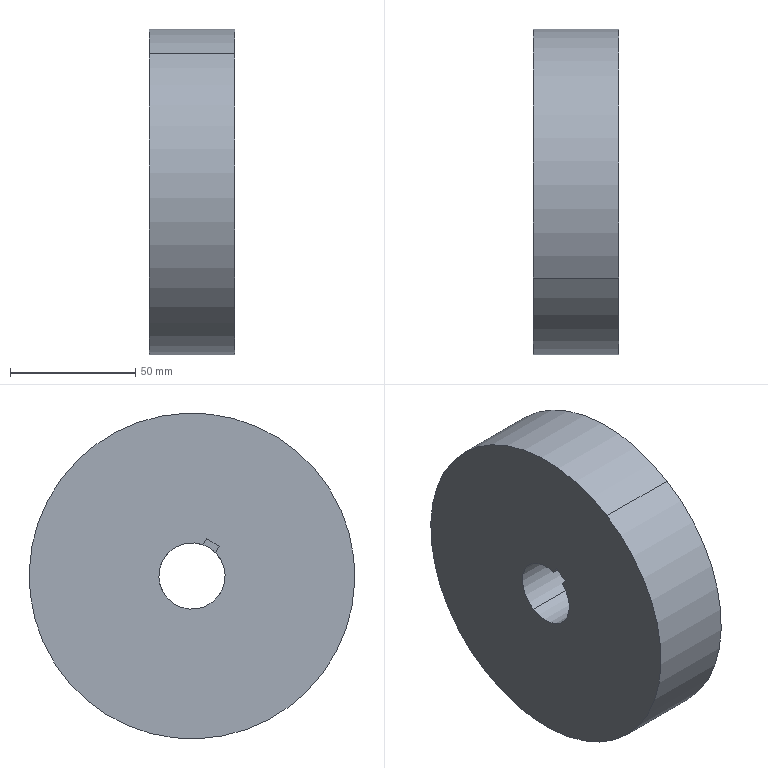Component | SolidWorks | Handwheel-1 | 1 solid | 13 faces | box 34 x 130 x 130 mm | volume 431777 mm3 | plane 7 | cylinder 6 | commonest cylinder face diameters 10 x2 26.469 x2 130 x2
build123d program:
from build123d import *

# Parameters (mm, degrees)
SKETCH1_R           = 65
SKETCH1_R_2         = 13.235
BOSS_EXTRUDE1_DEPTH = 34
SKETCH2_R           = 5
CUT_EXTRUDE1_DEPTH  = 8
CUT_EXTRUDE2_START  = -23
CUT_EXTRUDE2_DEPTH  = 11


with BuildPart() as part:
    # Sketch1 → Boss-Extrude1 (new body)
    with BuildSketch(Plane.XY):
        with Locations((15, 150)):
            Circle(SKETCH1_R)
        with Locations((15, 150)):
            Circle(SKETCH1_R_2, mode=Mode.SUBTRACT)
    extrude(amount=BOSS_EXTRUDE1_DEPTH)

    # Sketch2 → Cut-Extrude1 (cut)
    with BuildSketch(Plane.XY.offset(34)):
        with Locations((15, 199.291)):
            Circle(SKETCH2_R)
    extrude(amount=-CUT_EXTRUDE1_DEPTH, mode=Mode.SUBTRACT)

    # Sketch3 → Cut-Extrude2 (cut)
    with BuildSketch(Plane.XY.offset(34).offset(CUT_EXTRUDE2_START)):
        Polygon((2.855, 152.957), (-0.8059, 152.957), (-0.8059, 147.031), (2.855, 147.043), align=None)
    extrude(amount=-CUT_EXTRUDE2_DEPTH, mode=Mode.SUBTRACT)


solid = part.part

# Placed as in the assembly
solid = solid.moved(Location((133.63, 14.821, -81.721), (31.981, 90, 0)))
STEP:
#1=COLOUR_RGB('',0.7922,0.8196,0.9333);
#2=FILL_AREA_STYLE_COLOUR('',#1);
#3=FILL_AREA_STYLE('',(#2));
#4=SURFACE_STYLE_FILL_AREA(#3);
#5=SURFACE_SIDE_STYLE('',(#4));
#6=SURFACE_STYLE_USAGE(.BOTH.,#5);
#7=PRESENTATION_STYLE_ASSIGNMENT((#6));
#8=CARTESIAN_POINT('',(6.285,7.447,0.6042));
#9=VERTEX_POINT('',#8);
#10=CARTESIAN_POINT('',(6.285,7.656,0.2703));
#11=VERTEX_POINT('',#10);
#12=CARTESIAN_POINT('',(6.285,7.552,0.4372));
#13=DIRECTION('',(1.,0.,0.));
#14=DIRECTION('',(0.,0.5296,-0.8482));
#15=AXIS2_PLACEMENT_3D('',#12,#13,#14);
#16=CIRCLE('',#15,0.1969);
#17=EDGE_CURVE('',#9,#11,#16,.T.);
#18=ORIENTED_EDGE('',*,*,#17,.F.);
#19=CARTESIAN_POINT('',(6.6,7.447,0.6042));
#20=VERTEX_POINT('',#19);
#21=CARTESIAN_POINT('',(6.285,7.447,0.6042));
#22=DIRECTION('',(1.,0.,0.));
#23=VECTOR('',#22,39.37);
#24=LINE('',#21,#23);
#25=EDGE_CURVE('',#9,#20,#24,.T.);
#26=ORIENTED_EDGE('',*,*,#25,.T.);
#27=CARTESIAN_POINT('',(6.6,7.656,0.2703));
#28=VERTEX_POINT('',#27);
#29=CARTESIAN_POINT('',(6.6,7.552,0.4372));
#30=DIRECTION('',(1.,0.,0.));
#31=DIRECTION('',(0.,0.5296,-0.8482));
#32=AXIS2_PLACEMENT_3D('',#29,#30,#31);
#33=CIRCLE('',#32,0.1969);
#34=EDGE_CURVE('',#20,#28,#33,.T.);
#35=ORIENTED_EDGE('',*,*,#34,.T.);
#36=CARTESIAN_POINT('',(6.285,7.656,0.2703));
#37=DIRECTION('',(1.,0.,0.));
#38=VECTOR('',#37,39.37);
#39=LINE('',#36,#38);
#40=EDGE_CURVE('',#11,#28,#39,.T.);
#41=ORIENTED_EDGE('',*,*,#40,.F.);
#42=EDGE_LOOP('',(#18,#26,#35,#41));
#43=FACE_OUTER_BOUND('',#42,.T.);
#44=CARTESIAN_POINT('',(6.285,7.552,0.4372));
#45=DIRECTION('',(1.,0.,0.));
#46=DIRECTION('',(0.,0.5296,-0.8482));
#47=AXIS2_PLACEMENT_3D('',#44,#45,#46);
#48=CYLINDRICAL_SURFACE('',#47,0.1969);
#49=ADVANCED_FACE('',(#43),#48,.F.);
#50=CARTESIAN_POINT('',(6.6,5.63,-0.1486));
#51=VERTEX_POINT('',#50);
#52=CARTESIAN_POINT('',(6.6,6.181,-1.033));
#53=VERTEX_POINT('',#52);
#54=CARTESIAN_POINT('',(6.6,5.906,-0.5906));
#55=DIRECTION('',(1.,0.,0.));
#56=DIRECTION('',(0.,0.5296,-0.8482));
#57=AXIS2_PLACEMENT_3D('',#54,#55,#56);
#58=CIRCLE('',#57,0.5211);
#59=EDGE_CURVE('',#51,#53,#58,.T.);
#60=ORIENTED_EDGE('',*,*,#59,.T.);
#61=CARTESIAN_POINT('',(5.261,6.181,-1.033));
#62=VERTEX_POINT('',#61);
#63=CARTESIAN_POINT('',(6.6,6.181,-1.033));
#64=DIRECTION('',(-1.,-0.,-0.));
#65=VECTOR('',#64,39.37);
#66=LINE('',#63,#65);
#67=EDGE_CURVE('',#53,#62,#66,.T.);
#68=ORIENTED_EDGE('',*,*,#67,.T.);
#69=CARTESIAN_POINT('',(5.261,5.538,-0.2215));
#70=VERTEX_POINT('',#69);
#71=CARTESIAN_POINT('',(5.261,5.906,-0.5906));
#72=DIRECTION('',(1.,0.,0.));
#73=DIRECTION('',(0.,0.5296,-0.8482));
#74=AXIS2_PLACEMENT_3D('',#71,#72,#73);
#75=CIRCLE('',#74,0.5211);
#76=EDGE_CURVE('',#70,#62,#75,.T.);
#77=ORIENTED_EDGE('',*,*,#76,.F.);
#78=CARTESIAN_POINT('',(5.694,5.538,-0.2215));
#79=VERTEX_POINT('',#78);
#80=CARTESIAN_POINT('',(6.6,5.538,-0.2215));
#81=DIRECTION('',(-1.,-0.,-0.));
#82=VECTOR('',#81,39.37);
#83=LINE('',#80,#82);
#84=EDGE_CURVE('',#79,#70,#83,.T.);
#85=ORIENTED_EDGE('',*,*,#84,.F.);
#86=CARTESIAN_POINT('',(5.694,5.63,-0.1486));
#87=VERTEX_POINT('',#86);
#88=CARTESIAN_POINT('',(5.694,5.906,-0.5906));
#89=DIRECTION('',(-1.,-0.,-0.));
#90=DIRECTION('',(0.,-0.5296,0.8482));
#91=AXIS2_PLACEMENT_3D('',#88,#89,#90);
#92=CIRCLE('',#91,0.5211);
#93=EDGE_CURVE('',#79,#87,#92,.T.);
#94=ORIENTED_EDGE('',*,*,#93,.T.);
#95=CARTESIAN_POINT('',(6.6,5.63,-0.1486));
#96=DIRECTION('',(-1.,-0.,-0.));
#97=VECTOR('',#96,39.37);
#98=LINE('',#95,#97);
#99=EDGE_CURVE('',#51,#87,#98,.T.);
#100=ORIENTED_EDGE('',*,*,#99,.F.);
#101=EDGE_LOOP('',(#60,#68,#77,#85,#94,#100));
#102=FACE_OUTER_BOUND('',#101,.T.);
#103=CARTESIAN_POINT('',(6.6,5.906,-0.5906));
#104=DIRECTION('',(-1.,-0.,-0.));
#105=DIRECTION('',(0.,-0.5296,0.8482));
#106=AXIS2_PLACEMENT_3D('',#103,#104,#105);
#107=CYLINDRICAL_SURFACE('',#106,0.5211);
#108=ADVANCED_FACE('',(#102),#107,.F.);
#109=CARTESIAN_POINT('',(6.6,7.261,-2.761));
#110=VERTEX_POINT('',#109);
#111=CARTESIAN_POINT('',(6.6,4.55,1.58));
#112=VERTEX_POINT('',#111);
#113=CARTESIAN_POINT('',(6.6,5.906,-0.5906));
#114=DIRECTION('',(1.,0.,0.));
#115=DIRECTION('',(0.,0.5296,-0.8482));
#116=AXIS2_PLACEMENT_3D('',#113,#114,#115);
#117=CIRCLE('',#116,2.559);
#118=EDGE_CURVE('',#110,#112,#117,.T.);
#119=ORIENTED_EDGE('',*,*,#118,.F.);
#120=CARTESIAN_POINT('',(5.261,7.261,-2.761));
#121=VERTEX_POINT('',#120);
#122=CARTESIAN_POINT('',(6.6,7.261,-2.761));
#123=DIRECTION('',(-1.,-0.,-0.));
#124=VECTOR('',#123,39.37);
#125=LINE('',#122,#124);
#126=EDGE_CURVE('',#110,#121,#125,.T.);
#127=ORIENTED_EDGE('',*,*,#126,.T.);
#128=CARTESIAN_POINT('',(5.261,4.55,1.58));
#129=VERTEX_POINT('',#128);
#130=CARTESIAN_POINT('',(5.261,5.906,-0.5906));
#131=DIRECTION('',(1.,0.,0.));
#132=DIRECTION('',(0.,0.5296,-0.8482));
#133=AXIS2_PLACEMENT_3D('',#130,#131,#132);
#134=CIRCLE('',#133,2.559);
#135=EDGE_CURVE('',#121,#129,#134,.T.);
#136=ORIENTED_EDGE('',*,*,#135,.T.);
#137=CARTESIAN_POINT('',(6.6,4.55,1.58));
#138=DIRECTION('',(-1.,-0.,-0.));
#139=VECTOR('',#138,39.37);
#140=LINE('',#137,#139);
#141=EDGE_CURVE('',#112,#129,#140,.T.);
#142=ORIENTED_EDGE('',*,*,#141,.F.);
#143=EDGE_LOOP('',(#119,#127,#136,#142));
#144=FACE_OUTER_BOUND('',#143,.T.);
#145=CARTESIAN_POINT('',(6.6,5.906,-0.5906));
#146=DIRECTION('',(-1.,-0.,-0.));
#147=DIRECTION('',(0.,-0.5296,0.8482));
#148=AXIS2_PLACEMENT_3D('',#145,#146,#147);
#149=CYLINDRICAL_SURFACE('',#148,2.559);
#150=ADVANCED_FACE('',(#144),#149,.T.);
#151=CARTESIAN_POINT('',(6.6,7.552,0.4372));
#152=DIRECTION('',(1.,0.,0.));
#153=DIRECTION('',(0.,0.5296,-0.8482));
#154=AXIS2_PLACEMENT_3D('',#151,#152,#153);
#155=CIRCLE('',#154,0.1969);
#156=EDGE_CURVE('',#28,#20,#155,.T.);
#157=ORIENTED_EDGE('',*,*,#156,.F.);
#158=ORIENTED_EDGE('',*,*,#34,.F.);
#159=EDGE_LOOP('',(#157,#158));
#160=FACE_BOUND('',#159,.T.);
#161=CARTESIAN_POINT('',(6.6,5.906,-0.5906));
#162=DIRECTION('',(1.,0.,0.));
#163=DIRECTION('',(0.,0.5296,-0.8482));
#164=AXIS2_PLACEMENT_3D('',#161,#162,#163);
#165=CIRCLE('',#164,2.559);
#166=EDGE_CURVE('',#112,#110,#165,.T.);
#167=ORIENTED_EDGE('',*,*,#166,.T.);
#168=ORIENTED_EDGE('',*,*,#118,.T.);
#169=EDGE_LOOP('',(#167,#168));
#170=FACE_OUTER_BOUND('',#169,.T.);
#171=ORIENTED_EDGE('',*,*,#59,.F.);
#172=CARTESIAN_POINT('',(6.6,5.906,-0.5906));
#173=DIRECTION('',(1.,0.,0.));
#174=DIRECTION('',(0.,0.5296,-0.8482));
#175=AXIS2_PLACEMENT_3D('',#172,#173,#174);
#176=CIRCLE('',#175,0.5211);
#177=EDGE_CURVE('',#53,#51,#176,.T.);
#178=ORIENTED_EDGE('',*,*,#177,.F.);
#179=EDGE_LOOP('',(#171,#178));
#180=FACE_BOUND('',#179,.T.);
#181=CARTESIAN_POINT('',(6.6,5.906,-0.5906));
#182=DIRECTION('',(1.,0.,0.));
#183=DIRECTION('',(0.,0.5296,-0.8482));
#184=AXIS2_PLACEMENT_3D('',#181,#182,#183);
#185=PLANE('',#184);
#186=ADVANCED_FACE('',(#160,#170,#180),#185,.T.);
#187=CARTESIAN_POINT('',(5.261,5.906,-0.5906));
#188=DIRECTION('',(1.,0.,0.));
#189=DIRECTION('',(0.,0.5296,-0.8482));
#190=AXIS2_PLACEMENT_3D('',#187,#188,#189);
#191=CIRCLE('',#190,2.559);
#192=EDGE_CURVE('',#129,#121,#191,.T.);
#193=ORIENTED_EDGE('',*,*,#192,.F.);
#194=ORIENTED_EDGE('',*,*,#135,.F.);
#195=EDGE_LOOP('',(#193,#194));
#196=FACE_OUTER_BOUND('',#195,.T.);
#197=CARTESIAN_POINT('',(5.261,5.675,-0.001053));
#198=VERTEX_POINT('',#197);
#199=CARTESIAN_POINT('',(5.261,5.477,-0.1246));
#200=VERTEX_POINT('',#199);
#201=CARTESIAN_POINT('',(5.261,5.675,-0.001053));
#202=DIRECTION('',(0.,-0.8482,-0.5296));
#203=VECTOR('',#202,39.37);
#204=LINE('',#201,#203);
#205=EDGE_CURVE('',#198,#200,#204,.T.);
#206=ORIENTED_EDGE('',*,*,#205,.T.);
#207=CARTESIAN_POINT('',(5.261,5.477,-0.1246));
#208=DIRECTION('',(0.,0.5324,-0.8465));
#209=VECTOR('',#208,39.37);
#210=LINE('',#207,#209);
#211=EDGE_CURVE('',#200,#70,#210,.T.);
#212=ORIENTED_EDGE('',*,*,#211,.T.);
#213=ORIENTED_EDGE('',*,*,#76,.T.);
#214=CARTESIAN_POINT('',(5.261,5.735,-0.09809));
#215=VERTEX_POINT('',#214);
#216=CARTESIAN_POINT('',(5.261,5.906,-0.5906));
#217=DIRECTION('',(1.,0.,0.));
#218=DIRECTION('',(0.,0.5296,-0.8482));
#219=AXIS2_PLACEMENT_3D('',#216,#217,#218);
#220=CIRCLE('',#219,0.5211);
#221=EDGE_CURVE('',#62,#215,#220,.T.);
#222=ORIENTED_EDGE('',*,*,#221,.T.);
#223=CARTESIAN_POINT('',(5.261,5.751,-0.1233));
#224=DIRECTION('',(-0.,-0.5296,0.8482));
#225=VECTOR('',#224,39.37);
#226=LINE('',#223,#225);
#227=EDGE_CURVE('',#215,#198,#226,.T.);
#228=ORIENTED_EDGE('',*,*,#227,.T.);
#229=EDGE_LOOP('',(#206,#212,#213,#222,#228));
#230=FACE_BOUND('',#229,.T.);
#231=CARTESIAN_POINT('',(5.261,5.906,-0.5906));
#232=DIRECTION('',(1.,0.,0.));
#233=DIRECTION('',(0.,0.5296,-0.8482));
#234=AXIS2_PLACEMENT_3D('',#231,#232,#233);
#235=PLANE('',#234);
#236=ADVANCED_FACE('',(#196,#230),#235,.F.);
#237=ORIENTED_EDGE('',*,*,#126,.F.);
#238=ORIENTED_EDGE('',*,*,#166,.F.);
#239=ORIENTED_EDGE('',*,*,#141,.T.);
#240=ORIENTED_EDGE('',*,*,#192,.T.);
#241=EDGE_LOOP('',(#237,#238,#239,#240));
#242=FACE_OUTER_BOUND('',#241,.T.);
#243=CARTESIAN_POINT('',(6.6,5.906,-0.5906));
#244=DIRECTION('',(-1.,-0.,-0.));
#245=DIRECTION('',(0.,-0.5296,0.8482));
#246=AXIS2_PLACEMENT_3D('',#243,#244,#245);
#247=CYLINDRICAL_SURFACE('',#246,2.559);
#248=ADVANCED_FACE('',(#242),#247,.T.);
#249=ORIENTED_EDGE('',*,*,#67,.F.);
#250=ORIENTED_EDGE('',*,*,#177,.T.);
#251=ORIENTED_EDGE('',*,*,#99,.T.);
#252=CARTESIAN_POINT('',(5.694,5.735,-0.09809));
#253=VERTEX_POINT('',#252);
#254=CARTESIAN_POINT('',(5.694,5.906,-0.5906));
#255=DIRECTION('',(-1.,-0.,-0.));
#256=DIRECTION('',(0.,-0.5296,0.8482));
#257=AXIS2_PLACEMENT_3D('',#254,#255,#256);
#258=CIRCLE('',#257,0.5211);
#259=EDGE_CURVE('',#87,#253,#258,.T.);
#260=ORIENTED_EDGE('',*,*,#259,.T.);
#261=CARTESIAN_POINT('',(6.6,5.735,-0.09809));
#262=DIRECTION('',(1.,0.,0.));
#263=VECTOR('',#262,39.37);
#264=LINE('',#261,#263);
#265=EDGE_CURVE('',#215,#253,#264,.T.);
#266=ORIENTED_EDGE('',*,*,#265,.F.);
#267=ORIENTED_EDGE('',*,*,#221,.F.);
#268=EDGE_LOOP('',(#249,#250,#251,#260,#266,#267));
#269=FACE_OUTER_BOUND('',#268,.T.);
#270=CARTESIAN_POINT('',(6.6,5.906,-0.5906));
#271=DIRECTION('',(-1.,-0.,-0.));
#272=DIRECTION('',(0.,-0.5296,0.8482));
#273=AXIS2_PLACEMENT_3D('',#270,#271,#272);
#274=CYLINDRICAL_SURFACE('',#273,0.5211);
#275=ADVANCED_FACE('',(#269),#274,.F.);
#276=ORIENTED_EDGE('',*,*,#25,.F.);
#277=CARTESIAN_POINT('',(6.285,7.552,0.4372));
#278=DIRECTION('',(1.,0.,0.));
#279=DIRECTION('',(0.,0.5296,-0.8482));
#280=AXIS2_PLACEMENT_3D('',#277,#278,#279);
#281=CIRCLE('',#280,0.1969);
#282=EDGE_CURVE('',#11,#9,#281,.T.);
#283=ORIENTED_EDGE('',*,*,#282,.F.);
#284=ORIENTED_EDGE('',*,*,#40,.T.);
#285=ORIENTED_EDGE('',*,*,#156,.T.);
#286=EDGE_LOOP('',(#276,#283,#284,#285));
#287=FACE_OUTER_BOUND('',#286,.T.);
#288=CARTESIAN_POINT('',(6.285,7.552,0.4372));
#289=DIRECTION('',(1.,0.,0.));
#290=DIRECTION('',(0.,0.5296,-0.8482));
#291=AXIS2_PLACEMENT_3D('',#288,#289,#290);
#292=CYLINDRICAL_SURFACE('',#291,0.1969);
#293=ADVANCED_FACE('',(#287),#292,.F.);
#294=ORIENTED_EDGE('',*,*,#282,.T.);
#295=ORIENTED_EDGE('',*,*,#17,.T.);
#296=EDGE_LOOP('',(#294,#295));
#297=FACE_OUTER_BOUND('',#296,.T.);
#298=CARTESIAN_POINT('',(6.285,7.552,0.4372));
#299=DIRECTION('',(1.,0.,0.));
#300=DIRECTION('',(0.,0.5296,-0.8482));
#301=AXIS2_PLACEMENT_3D('',#298,#299,#300);
#302=PLANE('',#301);
#303=ADVANCED_FACE('',(#297),#302,.T.);
#304=ORIENTED_EDGE('',*,*,#84,.T.);
#305=ORIENTED_EDGE('',*,*,#211,.F.);
#306=CARTESIAN_POINT('',(5.694,5.477,-0.1246));
#307=VERTEX_POINT('',#306);
#308=CARTESIAN_POINT('',(5.261,5.477,-0.1246));
#309=DIRECTION('',(1.,0.,0.));
#310=VECTOR('',#309,39.37);
#311=LINE('',#308,#310);
#312=EDGE_CURVE('',#200,#307,#311,.T.);
#313=ORIENTED_EDGE('',*,*,#312,.T.);
#314=CARTESIAN_POINT('',(5.694,5.477,-0.1246));
#315=DIRECTION('',(0.,0.5324,-0.8465));
#316=VECTOR('',#315,39.37);
#317=LINE('',#314,#316);
#318=EDGE_CURVE('',#307,#79,#317,.T.);
#319=ORIENTED_EDGE('',*,*,#318,.T.);
#320=EDGE_LOOP('',(#304,#305,#313,#319));
#321=FACE_OUTER_BOUND('',#320,.T.);
#322=CARTESIAN_POINT('',(5.261,5.477,-0.1246));
#323=DIRECTION('',(0.,-0.8465,-0.5324));
#324=DIRECTION('',(0.,0.5324,-0.8465));
#325=AXIS2_PLACEMENT_3D('',#322,#323,#324);
#326=PLANE('',#325);
#327=ADVANCED_FACE('',(#321),#326,.F.);
#328=CARTESIAN_POINT('',(5.694,5.675,-0.001053));
#329=VERTEX_POINT('',#328);
#330=CARTESIAN_POINT('',(5.694,5.675,-0.001053));
#331=DIRECTION('',(0.,-0.8482,-0.5296));
#332=VECTOR('',#331,39.37);
#333=LINE('',#330,#332);
#334=EDGE_CURVE('',#329,#307,#333,.T.);
#335=ORIENTED_EDGE('',*,*,#334,.T.);
#336=ORIENTED_EDGE('',*,*,#312,.F.);
#337=ORIENTED_EDGE('',*,*,#205,.F.);
#338=CARTESIAN_POINT('',(5.261,5.675,-0.001053));
#339=DIRECTION('',(1.,0.,0.));
#340=VECTOR('',#339,39.37);
#341=LINE('',#338,#340);
#342=EDGE_CURVE('',#198,#329,#341,.T.);
#343=ORIENTED_EDGE('',*,*,#342,.T.);
#344=EDGE_LOOP('',(#335,#336,#337,#343));
#345=FACE_OUTER_BOUND('',#344,.T.);
#346=CARTESIAN_POINT('',(5.261,5.675,-0.001053));
#347=DIRECTION('',(-0.,-0.5296,0.8482));
#348=DIRECTION('',(1.,0.,0.));
#349=AXIS2_PLACEMENT_3D('',#346,#347,#348);
#350=PLANE('',#349);
#351=ADVANCED_FACE('',(#345),#350,.F.);
#352=ORIENTED_EDGE('',*,*,#265,.T.);
#353=CARTESIAN_POINT('',(5.694,5.751,-0.1233));
#354=DIRECTION('',(-0.,-0.5296,0.8482));
#355=VECTOR('',#354,39.37);
#356=LINE('',#353,#355);
#357=EDGE_CURVE('',#253,#329,#356,.T.);
#358=ORIENTED_EDGE('',*,*,#357,.T.);
#359=ORIENTED_EDGE('',*,*,#342,.F.);
#360=ORIENTED_EDGE('',*,*,#227,.F.);
#361=EDGE_LOOP('',(#352,#358,#359,#360));
#362=FACE_OUTER_BOUND('',#361,.T.);
#363=CARTESIAN_POINT('',(5.261,5.751,-0.1233));
#364=DIRECTION('',(-0.,0.8482,0.5296));
#365=DIRECTION('',(1.,0.,0.));
#366=AXIS2_PLACEMENT_3D('',#363,#364,#365);
#367=PLANE('',#366);
#368=ADVANCED_FACE('',(#362),#367,.F.);
#369=ORIENTED_EDGE('',*,*,#318,.F.);
#370=ORIENTED_EDGE('',*,*,#334,.F.);
#371=ORIENTED_EDGE('',*,*,#357,.F.);
#372=ORIENTED_EDGE('',*,*,#259,.F.);
#373=ORIENTED_EDGE('',*,*,#93,.F.);
#374=EDGE_LOOP('',(#369,#370,#371,#372,#373));
#375=FACE_OUTER_BOUND('',#374,.T.);
#376=CARTESIAN_POINT('',(5.694,0.5835,-3.217));
#377=DIRECTION('',(-1.,-0.,-0.));
#378=DIRECTION('',(-0.,-0.5296,0.8482));
#379=AXIS2_PLACEMENT_3D('',#376,#377,#378);
#380=PLANE('',#379);
#381=ADVANCED_FACE('',(#375),#380,.T.);
#382=CLOSED_SHELL('',(#49,#108,#150,#186,#236,#248,#275,#293,#303,#327,#351,#368,#381));
#383=MANIFOLD_SOLID_BREP('',#382);
#384=STYLED_ITEM('',(#7),#383);
#385=PRESENTATION_LAYER_ASSIGNMENT('','',(#384));
#386=(LENGTH_UNIT()NAMED_UNIT(*)SI_UNIT($,.METRE.));
#387=LENGTH_MEASURE_WITH_UNIT(LENGTH_MEASURE(0.0254),#386);
#388=DIMENSIONAL_EXPONENTS(1.,0.,0.,0.,0.,0.,0.);
#389=(CONVERSION_BASED_UNIT('',#387)LENGTH_UNIT()NAMED_UNIT(#388));
#390=UNCERTAINTY_MEASURE_WITH_UNIT(LENGTH_MEASURE(0.00001),#389,'','');
#391=(NAMED_UNIT(*)PLANE_ANGLE_UNIT()SI_UNIT($,.RADIAN.));
#392=(NAMED_UNIT(*)SI_UNIT($,.STERADIAN.)SOLID_ANGLE_UNIT());
#393=(GEOMETRIC_REPRESENTATION_CONTEXT(3)GLOBAL_UNCERTAINTY_ASSIGNED_CONTEXT((#390))GLOBAL_UNIT_ASSIGNED_CONTEXT((#389,#391,#392))REPRESENTATION_CONTEXT('',''));
#394=MECHANICAL_DESIGN_GEOMETRIC_PRESENTATION_REPRESENTATION('',(#384),#393);
#395=CARTESIAN_POINT('',(0.,0.,0.));
#396=DIRECTION('',(0.,0.,1.));
#397=DIRECTION('',(1.,0.,0.));
#398=AXIS2_PLACEMENT_3D('',#395,#396,#397);
#399=(LENGTH_UNIT()NAMED_UNIT(*)SI_UNIT($,.METRE.));
#400=LENGTH_MEASURE_WITH_UNIT(LENGTH_MEASURE(0.0254),#399);
#401=DIMENSIONAL_EXPONENTS(1.,0.,0.,0.,0.,0.,0.);
#402=(CONVERSION_BASED_UNIT('',#400)LENGTH_UNIT()NAMED_UNIT(#401));
#403=UNCERTAINTY_MEASURE_WITH_UNIT(LENGTH_MEASURE(0.00001),#402,'','');
#404=(NAMED_UNIT(*)PLANE_ANGLE_UNIT()SI_UNIT($,.RADIAN.));
#405=(NAMED_UNIT(*)SI_UNIT($,.STERADIAN.)SOLID_ANGLE_UNIT());
#406=(GEOMETRIC_REPRESENTATION_CONTEXT(3)GLOBAL_UNCERTAINTY_ASSIGNED_CONTEXT((#403))GLOBAL_UNIT_ASSIGNED_CONTEXT((#402,#404,#405))REPRESENTATION_CONTEXT('',''));
#407=ADVANCED_BREP_SHAPE_REPRESENTATION('',(#383,#398),#406);